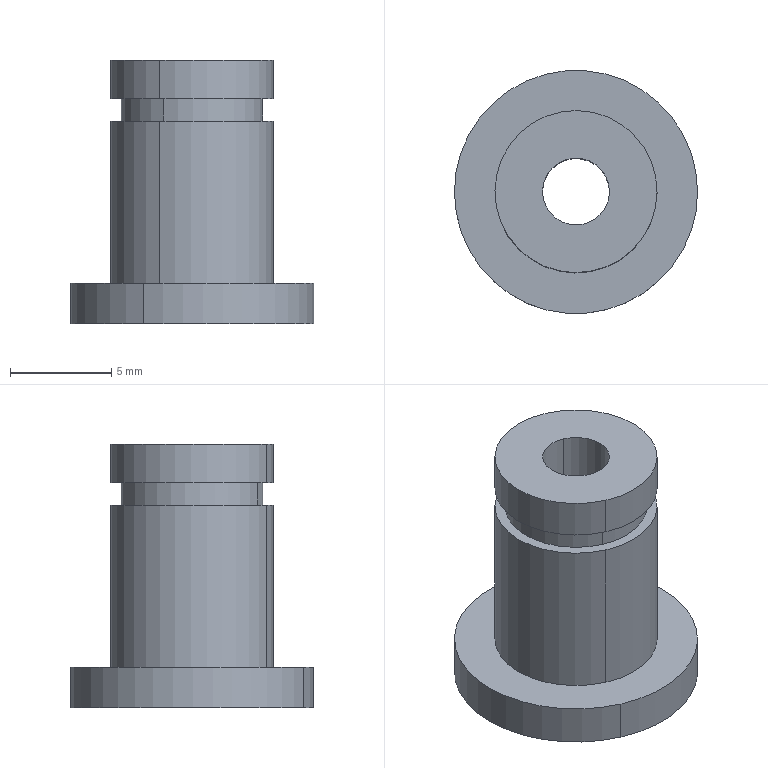Component | SolidWorks | PulleyAssembly-1_Axis-1 | 1 solid | 15 faces | box 12 x 12 x 13 mm | volume 655 mm3 | cylinder 10 | plane 5 | commonest cylinder face diameters 8 x4 7 x2 3.3 x2 12 x2
build123d program:
from build123d import *

# Parameters (mm, degrees)
SKETCH1_R              = 4
BOSS_EXTRUDE1_DEPTH    = 13
S2D0005_R              = 6
BOSS_EXTRUDE2_DEPTH    = 2
S2D0006_R              = 1.65
CUT_EXTRUDE1_DEPTH     = 14.3
SKETCH4_W              = 1.1
SKETCH4_H              = 0.5
CUT_SWEEP1_PITCH       = 0.7
CUT_SWEEP1_HEIGHT      = 0.5
CUT_SWEEP1_RADIUS      = 0.8477
CUT_SWEEP1_START_ANGLE = 179


with BuildPart() as part:
    # Sketch1 → Boss-Extrude1 (new body)
    with BuildSketch(Plane(origin=(0, 0, 0), x_dir=(1, 0, 0), z_dir=(0, 1, 0))):
        with Locations(Location((0, 0, 0), (0, 0, 90))):
            Circle(SKETCH1_R)
    extrude(amount=BOSS_EXTRUDE1_DEPTH)

    # S2D0005 → Boss-Extrude2 (add)
    with BuildSketch(Plane(origin=(0, 0, 0), x_dir=(0, 0, 1), z_dir=(0, -1, 0))):
        with Locations(Location((0, 0, 0), (0, 0, 180))):
            Circle(S2D0005_R)
    extrude(amount=-BOSS_EXTRUDE2_DEPTH)

    # S2D0006 → Cut-Extrude1 (cut)
    with BuildSketch(Plane(origin=(0, 13, 0), x_dir=(0, 0, -1), z_dir=(0, 1, 0))):
        with Locations(Location((0, 0, 0), (0, 0, 180))):
            Circle(S2D0006_R)
    extrude(amount=-CUT_EXTRUDE1_DEPTH, mode=Mode.SUBTRACT)

    # Sketch4 → Cut-Revolve1 (revolve, cut)
    with BuildSketch(Plane(origin=(0, 0, 0), x_dir=(0, -1, 0), z_dir=(0, 0, 1)), mode=Mode.PRIVATE) as cut_revolve1_sk:
        with Locations((-10.55, 3.75)):
            Rectangle(SKETCH4_W, SKETCH4_H)
    revolve(cut_revolve1_sk.sketch.rotate(Axis((0, 11.155, 0), (0, -1, 0)), 270), axis=Axis((0, 11.155, 0), (0, -1, 0)), mode=Mode.SUBTRACT)

    # Cut-Sweep1: sweep along a helix
    with BuildLine() as cut_sweep1_path:
        add(Helix(CUT_SWEEP1_PITCH, CUT_SWEEP1_HEIGHT, CUT_SWEEP1_RADIUS, center=(0, -1.65, -0.01459), direction=(0, -1, 0), mode=Mode.PRIVATE).rotate(Axis((0, -1.65, -0.01459), (0, -1, 0)), CUT_SWEEP1_START_ANGLE))
    # Sketch6 → Cut-Sweep1 (sweep, cut)
    with BuildSketch(Plane(origin=(0, 13.848, 1.65), x_dir=(0, 0, -1), z_dir=(-1, 0, 0))):
        Polygon((0, 0.25), (-0.433, 0), (0, -0.25), align=None)
    sweep(path=cut_sweep1_path.line, is_frenet=True, mode=Mode.SUBTRACT)


solid = part.part

# Placed as in the assembly
solid = solid.moved(Location((-354.55, -345.434, 483.481), (90, 0, 0)))
STEP:
#1=CARTESIAN_POINT('',(-14.013,-13.726,19.428));
#2=VERTEX_POINT('',#1);
#3=CARTESIAN_POINT('',(-13.904,-13.473,19.428));
#4=VERTEX_POINT('',#3);
#5=CARTESIAN_POINT('',(-13.959,-13.6,19.428));
#6=DIRECTION('',(0.,0.,1.));
#7=DIRECTION('',(-0.3954,-0.9185,0.));
#8=AXIS2_PLACEMENT_3D('',#5,#6,#7);
#9=CIRCLE('',#8,0.1378);
#10=EDGE_CURVE('',#2,#4,#9,.T.);
#11=ORIENTED_EDGE('',*,*,#10,.T.);
#12=CARTESIAN_POINT('',(-13.904,-13.473,19.472));
#13=VERTEX_POINT('',#12);
#14=CARTESIAN_POINT('',(-13.904,-13.473,19.474));
#15=DIRECTION('',(0.,0.,1.));
#16=VECTOR('',#15,39.37);
#17=LINE('',#14,#16);
#18=EDGE_CURVE('',#4,#13,#17,.T.);
#19=ORIENTED_EDGE('',*,*,#18,.T.);
#20=CARTESIAN_POINT('',(-14.013,-13.726,19.472));
#21=VERTEX_POINT('',#20);
#22=CARTESIAN_POINT('',(-13.959,-13.6,19.472));
#23=DIRECTION('',(0.,0.,1.));
#24=DIRECTION('',(-0.3954,-0.9185,0.));
#25=AXIS2_PLACEMENT_3D('',#22,#23,#24);
#26=CIRCLE('',#25,0.1378);
#27=EDGE_CURVE('',#21,#13,#26,.T.);
#28=ORIENTED_EDGE('',*,*,#27,.F.);
#29=CARTESIAN_POINT('',(-14.013,-13.726,19.474));
#30=DIRECTION('',(0.,0.,1.));
#31=VECTOR('',#30,39.37);
#32=LINE('',#29,#31);
#33=EDGE_CURVE('',#2,#21,#32,.T.);
#34=ORIENTED_EDGE('',*,*,#33,.F.);
#35=EDGE_LOOP('',(#11,#19,#28,#34));
#36=FACE_OUTER_BOUND('',#35,.T.);
#37=CARTESIAN_POINT('',(-13.959,-13.6,19.474));
#38=DIRECTION('',(0.,0.,1.));
#39=DIRECTION('',(-0.3954,-0.9185,0.));
#40=AXIS2_PLACEMENT_3D('',#37,#38,#39);
#41=CYLINDRICAL_SURFACE('',#40,0.1378);
#42=ADVANCED_FACE('',(#36),#41,.T.);
#43=CARTESIAN_POINT('',(-13.933,-13.54,19.035));
#44=VERTEX_POINT('',#43);
#45=CARTESIAN_POINT('',(-13.984,-13.659,19.035));
#46=VERTEX_POINT('',#45);
#47=CARTESIAN_POINT('',(-13.959,-13.6,19.035));
#48=DIRECTION('',(0.,0.,1.));
#49=DIRECTION('',(-0.3954,-0.9185,0.));
#50=AXIS2_PLACEMENT_3D('',#47,#48,#49);
#51=CIRCLE('',#50,0.06496);
#52=EDGE_CURVE('',#44,#46,#51,.T.);
#53=ORIENTED_EDGE('',*,*,#52,.F.);
#54=CARTESIAN_POINT('',(-13.933,-13.54,19.546));
#55=VERTEX_POINT('',#54);
#56=CARTESIAN_POINT('',(-13.933,-13.54,18.983));
#57=DIRECTION('',(0.,0.,1.));
#58=VECTOR('',#57,39.37);
#59=LINE('',#56,#58);
#60=EDGE_CURVE('',#44,#55,#59,.T.);
#61=ORIENTED_EDGE('',*,*,#60,.T.);
#62=CARTESIAN_POINT('',(-13.984,-13.659,19.546));
#63=VERTEX_POINT('',#62);
#64=CARTESIAN_POINT('',(-13.959,-13.6,19.546));
#65=DIRECTION('',(0.,0.,1.));
#66=DIRECTION('',(-0.3954,-0.9185,0.));
#67=AXIS2_PLACEMENT_3D('',#64,#65,#66);
#68=CIRCLE('',#67,0.06496);
#69=EDGE_CURVE('',#55,#63,#68,.T.);
#70=ORIENTED_EDGE('',*,*,#69,.T.);
#71=CARTESIAN_POINT('',(-13.984,-13.659,18.983));
#72=DIRECTION('',(0.,0.,1.));
#73=VECTOR('',#72,39.37);
#74=LINE('',#71,#73);
#75=EDGE_CURVE('',#46,#63,#74,.T.);
#76=ORIENTED_EDGE('',*,*,#75,.F.);
#77=EDGE_LOOP('',(#53,#61,#70,#76));
#78=FACE_OUTER_BOUND('',#77,.T.);
#79=CARTESIAN_POINT('',(-13.959,-13.6,18.983));
#80=DIRECTION('',(0.,0.,1.));
#81=DIRECTION('',(-0.3954,-0.9185,0.));
#82=AXIS2_PLACEMENT_3D('',#79,#80,#81);
#83=CYLINDRICAL_SURFACE('',#82,0.06496);
#84=ADVANCED_FACE('',(#78),#83,.F.);
#85=CARTESIAN_POINT('',(-13.865,-13.383,19.113));
#86=VERTEX_POINT('',#85);
#87=CARTESIAN_POINT('',(-14.052,-13.817,19.113));
#88=VERTEX_POINT('',#87);
#89=CARTESIAN_POINT('',(-13.959,-13.6,19.113));
#90=DIRECTION('',(0.,-0.,-1.));
#91=DIRECTION('',(0.3954,0.9185,0.));
#92=AXIS2_PLACEMENT_3D('',#89,#90,#91);
#93=CIRCLE('',#92,0.2362);
#94=EDGE_CURVE('',#86,#88,#93,.T.);
#95=ORIENTED_EDGE('',*,*,#94,.T.);
#96=CARTESIAN_POINT('',(-14.052,-13.817,19.035));
#97=VERTEX_POINT('',#96);
#98=CARTESIAN_POINT('',(-14.052,-13.817,19.113));
#99=DIRECTION('',(0.,-0.,-1.));
#100=VECTOR('',#99,39.37);
#101=LINE('',#98,#100);
#102=EDGE_CURVE('',#88,#97,#101,.T.);
#103=ORIENTED_EDGE('',*,*,#102,.T.);
#104=CARTESIAN_POINT('',(-13.865,-13.383,19.035));
#105=VERTEX_POINT('',#104);
#106=CARTESIAN_POINT('',(-13.959,-13.6,19.035));
#107=DIRECTION('',(0.,-0.,-1.));
#108=DIRECTION('',(0.3954,0.9185,0.));
#109=AXIS2_PLACEMENT_3D('',#106,#107,#108);
#110=CIRCLE('',#109,0.2362);
#111=EDGE_CURVE('',#105,#97,#110,.T.);
#112=ORIENTED_EDGE('',*,*,#111,.F.);
#113=CARTESIAN_POINT('',(-13.865,-13.383,19.113));
#114=DIRECTION('',(0.,-0.,-1.));
#115=VECTOR('',#114,39.37);
#116=LINE('',#113,#115);
#117=EDGE_CURVE('',#86,#105,#116,.T.);
#118=ORIENTED_EDGE('',*,*,#117,.F.);
#119=EDGE_LOOP('',(#95,#103,#112,#118));
#120=FACE_OUTER_BOUND('',#119,.T.);
#121=CARTESIAN_POINT('',(-13.959,-13.6,19.113));
#122=DIRECTION('',(0.,-0.,-1.));
#123=DIRECTION('',(0.3954,0.9185,0.));
#124=AXIS2_PLACEMENT_3D('',#121,#122,#123);
#125=CYLINDRICAL_SURFACE('',#124,0.2362);
#126=ADVANCED_FACE('',(#120),#125,.T.);
#127=CARTESIAN_POINT('',(-14.021,-13.744,19.428));
#128=VERTEX_POINT('',#127);
#129=CARTESIAN_POINT('',(-13.896,-13.455,19.428));
#130=VERTEX_POINT('',#129);
#131=CARTESIAN_POINT('',(-13.959,-13.6,19.428));
#132=DIRECTION('',(0.,0.,1.));
#133=DIRECTION('',(-0.3954,-0.9185,0.));
#134=AXIS2_PLACEMENT_3D('',#131,#132,#133);
#135=CIRCLE('',#134,0.1575);
#136=EDGE_CURVE('',#128,#130,#135,.T.);
#137=ORIENTED_EDGE('',*,*,#136,.F.);
#138=CARTESIAN_POINT('',(-14.021,-13.744,19.113));
#139=VERTEX_POINT('',#138);
#140=CARTESIAN_POINT('',(-14.021,-13.744,19.546));
#141=DIRECTION('',(0.,-0.,-1.));
#142=VECTOR('',#141,39.37);
#143=LINE('',#140,#142);
#144=EDGE_CURVE('',#128,#139,#143,.T.);
#145=ORIENTED_EDGE('',*,*,#144,.T.);
#146=CARTESIAN_POINT('',(-13.896,-13.455,19.113));
#147=VERTEX_POINT('',#146);
#148=CARTESIAN_POINT('',(-13.959,-13.6,19.113));
#149=DIRECTION('',(0.,-0.,-1.));
#150=DIRECTION('',(0.3954,0.9185,0.));
#151=AXIS2_PLACEMENT_3D('',#148,#149,#150);
#152=CIRCLE('',#151,0.1575);
#153=EDGE_CURVE('',#147,#139,#152,.T.);
#154=ORIENTED_EDGE('',*,*,#153,.F.);
#155=CARTESIAN_POINT('',(-13.896,-13.455,19.546));
#156=DIRECTION('',(0.,-0.,-1.));
#157=VECTOR('',#156,39.37);
#158=LINE('',#155,#157);
#159=EDGE_CURVE('',#130,#147,#158,.T.);
#160=ORIENTED_EDGE('',*,*,#159,.F.);
#161=EDGE_LOOP('',(#137,#145,#154,#160));
#162=FACE_OUTER_BOUND('',#161,.T.);
#163=CARTESIAN_POINT('',(-13.959,-13.6,19.546));
#164=DIRECTION('',(0.,-0.,-1.));
#165=DIRECTION('',(0.3954,0.9185,0.));
#166=AXIS2_PLACEMENT_3D('',#163,#164,#165);
#167=CYLINDRICAL_SURFACE('',#166,0.1575);
#168=ADVANCED_FACE('',(#162),#167,.T.);
#169=CARTESIAN_POINT('',(-14.021,-13.744,19.546));
#170=VERTEX_POINT('',#169);
#171=CARTESIAN_POINT('',(-13.896,-13.455,19.546));
#172=VERTEX_POINT('',#171);
#173=CARTESIAN_POINT('',(-13.959,-13.6,19.546));
#174=DIRECTION('',(0.,0.,1.));
#175=DIRECTION('',(-0.3954,-0.9185,0.));
#176=AXIS2_PLACEMENT_3D('',#173,#174,#175);
#177=CIRCLE('',#176,0.1575);
#178=EDGE_CURVE('',#170,#172,#177,.T.);
#179=ORIENTED_EDGE('',*,*,#178,.F.);
#180=CARTESIAN_POINT('',(-14.021,-13.744,19.472));
#181=VERTEX_POINT('',#180);
#182=CARTESIAN_POINT('',(-14.021,-13.744,19.546));
#183=DIRECTION('',(0.,-0.,-1.));
#184=VECTOR('',#183,39.37);
#185=LINE('',#182,#184);
#186=EDGE_CURVE('',#170,#181,#185,.T.);
#187=ORIENTED_EDGE('',*,*,#186,.T.);
#188=CARTESIAN_POINT('',(-13.896,-13.455,19.472));
#189=VERTEX_POINT('',#188);
#190=CARTESIAN_POINT('',(-13.959,-13.6,19.472));
#191=DIRECTION('',(0.,0.,1.));
#192=DIRECTION('',(-0.3954,-0.9185,0.));
#193=AXIS2_PLACEMENT_3D('',#190,#191,#192);
#194=CIRCLE('',#193,0.1575);
#195=EDGE_CURVE('',#181,#189,#194,.T.);
#196=ORIENTED_EDGE('',*,*,#195,.T.);
#197=CARTESIAN_POINT('',(-13.896,-13.455,19.546));
#198=DIRECTION('',(0.,-0.,-1.));
#199=VECTOR('',#198,39.37);
#200=LINE('',#197,#199);
#201=EDGE_CURVE('',#172,#189,#200,.T.);
#202=ORIENTED_EDGE('',*,*,#201,.F.);
#203=EDGE_LOOP('',(#179,#187,#196,#202));
#204=FACE_OUTER_BOUND('',#203,.T.);
#205=CARTESIAN_POINT('',(-13.959,-13.6,19.546));
#206=DIRECTION('',(0.,-0.,-1.));
#207=DIRECTION('',(0.3954,0.9185,0.));
#208=AXIS2_PLACEMENT_3D('',#205,#206,#207);
#209=CYLINDRICAL_SURFACE('',#208,0.1575);
#210=ADVANCED_FACE('',(#204),#209,.T.);
#211=ORIENTED_EDGE('',*,*,#186,.F.);
#212=CARTESIAN_POINT('',(-13.959,-13.6,19.546));
#213=DIRECTION('',(0.,0.,1.));
#214=DIRECTION('',(-0.3954,-0.9185,0.));
#215=AXIS2_PLACEMENT_3D('',#212,#213,#214);
#216=CIRCLE('',#215,0.1575);
#217=EDGE_CURVE('',#172,#170,#216,.T.);
#218=ORIENTED_EDGE('',*,*,#217,.F.);
#219=ORIENTED_EDGE('',*,*,#201,.T.);
#220=CARTESIAN_POINT('',(-13.959,-13.6,19.472));
#221=DIRECTION('',(0.,0.,1.));
#222=DIRECTION('',(-0.3954,-0.9185,0.));
#223=AXIS2_PLACEMENT_3D('',#220,#221,#222);
#224=CIRCLE('',#223,0.1575);
#225=EDGE_CURVE('',#189,#181,#224,.T.);
#226=ORIENTED_EDGE('',*,*,#225,.T.);
#227=EDGE_LOOP('',(#211,#218,#219,#226));
#228=FACE_OUTER_BOUND('',#227,.T.);
#229=CARTESIAN_POINT('',(-13.959,-13.6,19.546));
#230=DIRECTION('',(0.,-0.,-1.));
#231=DIRECTION('',(0.3954,0.9185,0.));
#232=AXIS2_PLACEMENT_3D('',#229,#230,#231);
#233=CYLINDRICAL_SURFACE('',#232,0.1575);
#234=ADVANCED_FACE('',(#228),#233,.T.);
#235=ORIENTED_EDGE('',*,*,#144,.F.);
#236=CARTESIAN_POINT('',(-13.959,-13.6,19.428));
#237=DIRECTION('',(0.,0.,1.));
#238=DIRECTION('',(-0.3954,-0.9185,0.));
#239=AXIS2_PLACEMENT_3D('',#236,#237,#238);
#240=CIRCLE('',#239,0.1575);
#241=EDGE_CURVE('',#130,#128,#240,.T.);
#242=ORIENTED_EDGE('',*,*,#241,.F.);
#243=ORIENTED_EDGE('',*,*,#159,.T.);
#244=CARTESIAN_POINT('',(-13.959,-13.6,19.113));
#245=DIRECTION('',(0.,-0.,-1.));
#246=DIRECTION('',(0.3954,0.9185,0.));
#247=AXIS2_PLACEMENT_3D('',#244,#245,#246);
#248=CIRCLE('',#247,0.1575);
#249=EDGE_CURVE('',#139,#147,#248,.T.);
#250=ORIENTED_EDGE('',*,*,#249,.F.);
#251=EDGE_LOOP('',(#235,#242,#243,#250));
#252=FACE_OUTER_BOUND('',#251,.T.);
#253=CARTESIAN_POINT('',(-13.959,-13.6,19.546));
#254=DIRECTION('',(0.,-0.,-1.));
#255=DIRECTION('',(0.3954,0.9185,0.));
#256=AXIS2_PLACEMENT_3D('',#253,#254,#255);
#257=CYLINDRICAL_SURFACE('',#256,0.1575);
#258=ADVANCED_FACE('',(#252),#257,.T.);
#259=CARTESIAN_POINT('',(-13.959,-13.6,19.546));
#260=DIRECTION('',(0.,0.,1.));
#261=DIRECTION('',(-0.3954,-0.9185,0.));
#262=AXIS2_PLACEMENT_3D('',#259,#260,#261);
#263=CIRCLE('',#262,0.06496);
#264=EDGE_CURVE('',#63,#55,#263,.T.);
#265=ORIENTED_EDGE('',*,*,#264,.F.);
#266=ORIENTED_EDGE('',*,*,#69,.F.);
#267=EDGE_LOOP('',(#265,#266));
#268=FACE_BOUND('',#267,.T.);
#269=ORIENTED_EDGE('',*,*,#217,.T.);
#270=ORIENTED_EDGE('',*,*,#178,.T.);
#271=EDGE_LOOP('',(#269,#270));
#272=FACE_OUTER_BOUND('',#271,.T.);
#273=CARTESIAN_POINT('',(-13.959,-13.6,19.546));
#274=DIRECTION('',(-0.,0.,1.));
#275=DIRECTION('',(-0.3954,-0.9185,0.));
#276=AXIS2_PLACEMENT_3D('',#273,#274,#275);
#277=PLANE('',#276);
#278=ADVANCED_FACE('',(#268,#272),#277,.T.);
#279=ORIENTED_EDGE('',*,*,#94,.F.);
#280=CARTESIAN_POINT('',(-13.959,-13.6,19.113));
#281=DIRECTION('',(0.,-0.,-1.));
#282=DIRECTION('',(0.3954,0.9185,0.));
#283=AXIS2_PLACEMENT_3D('',#280,#281,#282);
#284=CIRCLE('',#283,0.2362);
#285=EDGE_CURVE('',#88,#86,#284,.T.);
#286=ORIENTED_EDGE('',*,*,#285,.F.);
#287=EDGE_LOOP('',(#279,#286));
#288=FACE_OUTER_BOUND('',#287,.T.);
#289=ORIENTED_EDGE('',*,*,#153,.T.);
#290=ORIENTED_EDGE('',*,*,#249,.T.);
#291=EDGE_LOOP('',(#289,#290));
#292=FACE_BOUND('',#291,.T.);
#293=CARTESIAN_POINT('',(-13.959,-13.6,19.113));
#294=DIRECTION('',(0.,-0.,-1.));
#295=DIRECTION('',(0.3954,0.9185,-0.));
#296=AXIS2_PLACEMENT_3D('',#293,#294,#295);
#297=PLANE('',#296);
#298=ADVANCED_FACE('',(#288,#292),#297,.F.);
#299=ORIENTED_EDGE('',*,*,#102,.F.);
#300=ORIENTED_EDGE('',*,*,#285,.T.);
#301=ORIENTED_EDGE('',*,*,#117,.T.);
#302=CARTESIAN_POINT('',(-13.959,-13.6,19.035));
#303=DIRECTION('',(0.,-0.,-1.));
#304=DIRECTION('',(0.3954,0.9185,0.));
#305=AXIS2_PLACEMENT_3D('',#302,#303,#304);
#306=CIRCLE('',#305,0.2362);
#307=EDGE_CURVE('',#97,#105,#306,.T.);
#308=ORIENTED_EDGE('',*,*,#307,.F.);
#309=EDGE_LOOP('',(#299,#300,#301,#308));
#310=FACE_OUTER_BOUND('',#309,.T.);
#311=CARTESIAN_POINT('',(-13.959,-13.6,19.113));
#312=DIRECTION('',(0.,-0.,-1.));
#313=DIRECTION('',(0.3954,0.9185,0.));
#314=AXIS2_PLACEMENT_3D('',#311,#312,#313);
#315=CYLINDRICAL_SURFACE('',#314,0.2362);
#316=ADVANCED_FACE('',(#310),#315,.T.);
#317=CARTESIAN_POINT('',(-13.959,-13.6,19.035));
#318=DIRECTION('',(0.,0.,1.));
#319=DIRECTION('',(-0.3954,-0.9185,0.));
#320=AXIS2_PLACEMENT_3D('',#317,#318,#319);
#321=CIRCLE('',#320,0.06496);
#322=EDGE_CURVE('',#46,#44,#321,.T.);
#323=ORIENTED_EDGE('',*,*,#322,.T.);
#324=ORIENTED_EDGE('',*,*,#52,.T.);
#325=EDGE_LOOP('',(#323,#324));
#326=FACE_BOUND('',#325,.T.);
#327=ORIENTED_EDGE('',*,*,#111,.T.);
#328=ORIENTED_EDGE('',*,*,#307,.T.);
#329=EDGE_LOOP('',(#327,#328));
#330=FACE_OUTER_BOUND('',#329,.T.);
#331=CARTESIAN_POINT('',(-13.959,-13.6,19.035));
#332=DIRECTION('',(-0.,0.,1.));
#333=DIRECTION('',(-0.3954,-0.9185,0.));
#334=AXIS2_PLACEMENT_3D('',#331,#332,#333);
#335=PLANE('',#334);
#336=ADVANCED_FACE('',(#326,#330),#335,.F.);
#337=ORIENTED_EDGE('',*,*,#60,.F.);
#338=ORIENTED_EDGE('',*,*,#322,.F.);
#339=ORIENTED_EDGE('',*,*,#75,.T.);
#340=ORIENTED_EDGE('',*,*,#264,.T.);
#341=EDGE_LOOP('',(#337,#338,#339,#340));
#342=FACE_OUTER_BOUND('',#341,.T.);
#343=CARTESIAN_POINT('',(-13.959,-13.6,18.983));
#344=DIRECTION('',(0.,0.,1.));
#345=DIRECTION('',(-0.3954,-0.9185,0.));
#346=AXIS2_PLACEMENT_3D('',#343,#344,#345);
#347=CYLINDRICAL_SURFACE('',#346,0.06496);
#348=ADVANCED_FACE('',(#342),#347,.F.);
#349=ORIENTED_EDGE('',*,*,#27,.T.);
#350=CARTESIAN_POINT('',(-13.959,-13.6,19.472));
#351=DIRECTION('',(0.,0.,1.));
#352=DIRECTION('',(-0.3954,-0.9185,0.));
#353=AXIS2_PLACEMENT_3D('',#350,#351,#352);
#354=CIRCLE('',#353,0.1378);
#355=EDGE_CURVE('',#13,#21,#354,.T.);
#356=ORIENTED_EDGE('',*,*,#355,.T.);
#357=EDGE_LOOP('',(#349,#356));
#358=FACE_BOUND('',#357,.T.);
#359=ORIENTED_EDGE('',*,*,#225,.F.);
#360=ORIENTED_EDGE('',*,*,#195,.F.);
#361=EDGE_LOOP('',(#359,#360));
#362=FACE_OUTER_BOUND('',#361,.T.);
#363=CARTESIAN_POINT('',(-13.832,-13.654,19.472));
#364=DIRECTION('',(0.,-0.,-1.));
#365=DIRECTION('',(0.3954,0.9185,-0.));
#366=AXIS2_PLACEMENT_3D('',#363,#364,#365);
#367=PLANE('',#366);
#368=ADVANCED_FACE('',(#358,#362),#367,.T.);
#369=ORIENTED_EDGE('',*,*,#241,.T.);
#370=ORIENTED_EDGE('',*,*,#136,.T.);
#371=EDGE_LOOP('',(#369,#370));
#372=FACE_OUTER_BOUND('',#371,.T.);
#373=ORIENTED_EDGE('',*,*,#10,.F.);
#374=CARTESIAN_POINT('',(-13.959,-13.6,19.428));
#375=DIRECTION('',(0.,0.,1.));
#376=DIRECTION('',(-0.3954,-0.9185,0.));
#377=AXIS2_PLACEMENT_3D('',#374,#375,#376);
#378=CIRCLE('',#377,0.1378);
#379=EDGE_CURVE('',#4,#2,#378,.T.);
#380=ORIENTED_EDGE('',*,*,#379,.F.);
#381=EDGE_LOOP('',(#373,#380));
#382=FACE_BOUND('',#381,.T.);
#383=CARTESIAN_POINT('',(-13.814,-13.662,19.428));
#384=DIRECTION('',(-0.,0.,1.));
#385=DIRECTION('',(-0.3954,-0.9185,0.));
#386=AXIS2_PLACEMENT_3D('',#383,#384,#385);
#387=PLANE('',#386);
#388=ADVANCED_FACE('',(#372,#382),#387,.T.);
#389=ORIENTED_EDGE('',*,*,#18,.F.);
#390=ORIENTED_EDGE('',*,*,#379,.T.);
#391=ORIENTED_EDGE('',*,*,#33,.T.);
#392=ORIENTED_EDGE('',*,*,#355,.F.);
#393=EDGE_LOOP('',(#389,#390,#391,#392));
#394=FACE_OUTER_BOUND('',#393,.T.);
#395=CARTESIAN_POINT('',(-13.959,-13.6,19.474));
#396=DIRECTION('',(0.,0.,1.));
#397=DIRECTION('',(-0.3954,-0.9185,0.));
#398=AXIS2_PLACEMENT_3D('',#395,#396,#397);
#399=CYLINDRICAL_SURFACE('',#398,0.1378);
#400=ADVANCED_FACE('',(#394),#399,.T.);
#401=CLOSED_SHELL('',(#42,#84,#126,#168,#210,#234,#258,#278,#298,#316,#336,#348,#368,#388,#400));
#402=MANIFOLD_SOLID_BREP('',#401);
#403=CARTESIAN_POINT('',(0.,0.,0.));
#404=DIRECTION('',(0.,0.,1.));
#405=DIRECTION('',(1.,0.,0.));
#406=AXIS2_PLACEMENT_3D('',#403,#404,#405);
#407=(LENGTH_UNIT()NAMED_UNIT(*)SI_UNIT($,.METRE.));
#408=LENGTH_MEASURE_WITH_UNIT(LENGTH_MEASURE(0.0254),#407);
#409=DIMENSIONAL_EXPONENTS(1.,0.,0.,0.,0.,0.,0.);
#410=(CONVERSION_BASED_UNIT('',#408)LENGTH_UNIT()NAMED_UNIT(#409));
#411=UNCERTAINTY_MEASURE_WITH_UNIT(LENGTH_MEASURE(0.00001),#410,'','');
#412=(NAMED_UNIT(*)PLANE_ANGLE_UNIT()SI_UNIT($,.RADIAN.));
#413=(NAMED_UNIT(*)SI_UNIT($,.STERADIAN.)SOLID_ANGLE_UNIT());
#414=(GEOMETRIC_REPRESENTATION_CONTEXT(3)GLOBAL_UNCERTAINTY_ASSIGNED_CONTEXT((#411))GLOBAL_UNIT_ASSIGNED_CONTEXT((#410,#412,#413))REPRESENTATION_CONTEXT('',''));
#415=ADVANCED_BREP_SHAPE_REPRESENTATION('',(#402,#406),#414);
#416=COLOUR_RGB('',0.7922,0.8196,0.9333);
#417=FILL_AREA_STYLE_COLOUR('',#416);
#418=FILL_AREA_STYLE('',(#417));
#419=SURFACE_STYLE_FILL_AREA(#418);
#420=SURFACE_SIDE_STYLE('',(#419));
#421=SURFACE_STYLE_USAGE(.BOTH.,#420);
#422=PRESENTATION_STYLE_ASSIGNMENT((#421));
#423=STYLED_ITEM('',(#422),#402);
#424=(LENGTH_UNIT()NAMED_UNIT(*)SI_UNIT($,.METRE.));
#425=LENGTH_MEASURE_WITH_UNIT(LENGTH_MEASURE(0.0254),#424);
#426=DIMENSIONAL_EXPONENTS(1.,0.,0.,0.,0.,0.,0.);
#427=(CONVERSION_BASED_UNIT('',#425)LENGTH_UNIT()NAMED_UNIT(#426));
#428=UNCERTAINTY_MEASURE_WITH_UNIT(LENGTH_MEASURE(0.00001),#427,'','');
#429=(NAMED_UNIT(*)PLANE_ANGLE_UNIT()SI_UNIT($,.RADIAN.));
#430=(NAMED_UNIT(*)SI_UNIT($,.STERADIAN.)SOLID_ANGLE_UNIT());
#431=(GEOMETRIC_REPRESENTATION_CONTEXT(3)GLOBAL_UNCERTAINTY_ASSIGNED_CONTEXT((#428))GLOBAL_UNIT_ASSIGNED_CONTEXT((#427,#429,#430))REPRESENTATION_CONTEXT('',''));
#432=MECHANICAL_DESIGN_GEOMETRIC_PRESENTATION_REPRESENTATION('',(#423),#431);
#433=PRESENTATION_LAYER_ASSIGNMENT('','',(#423));